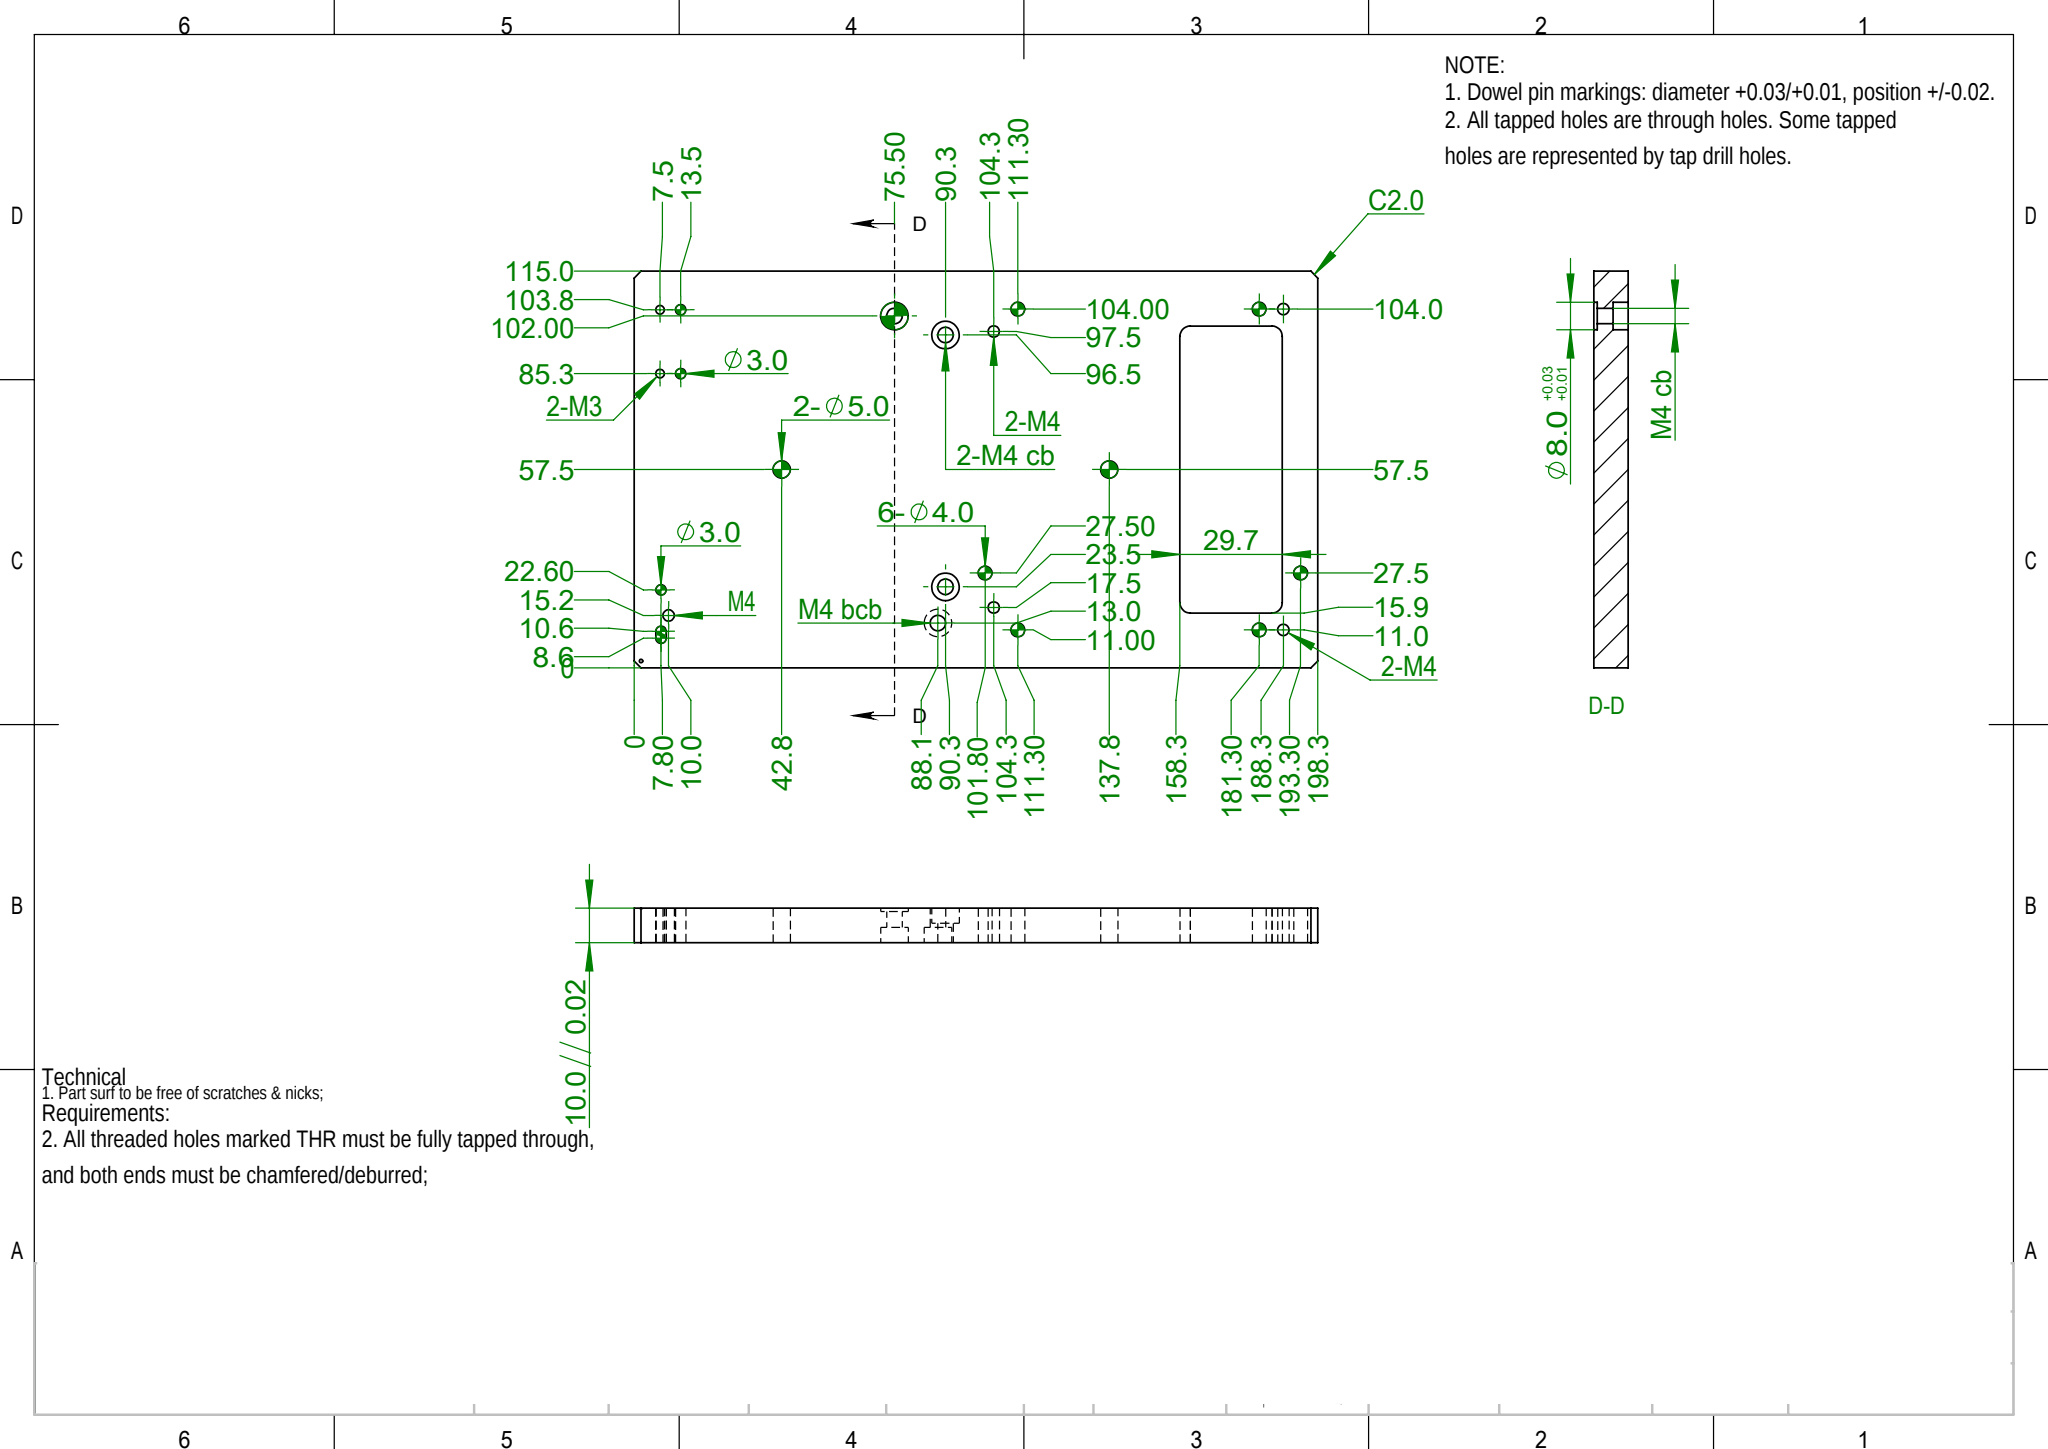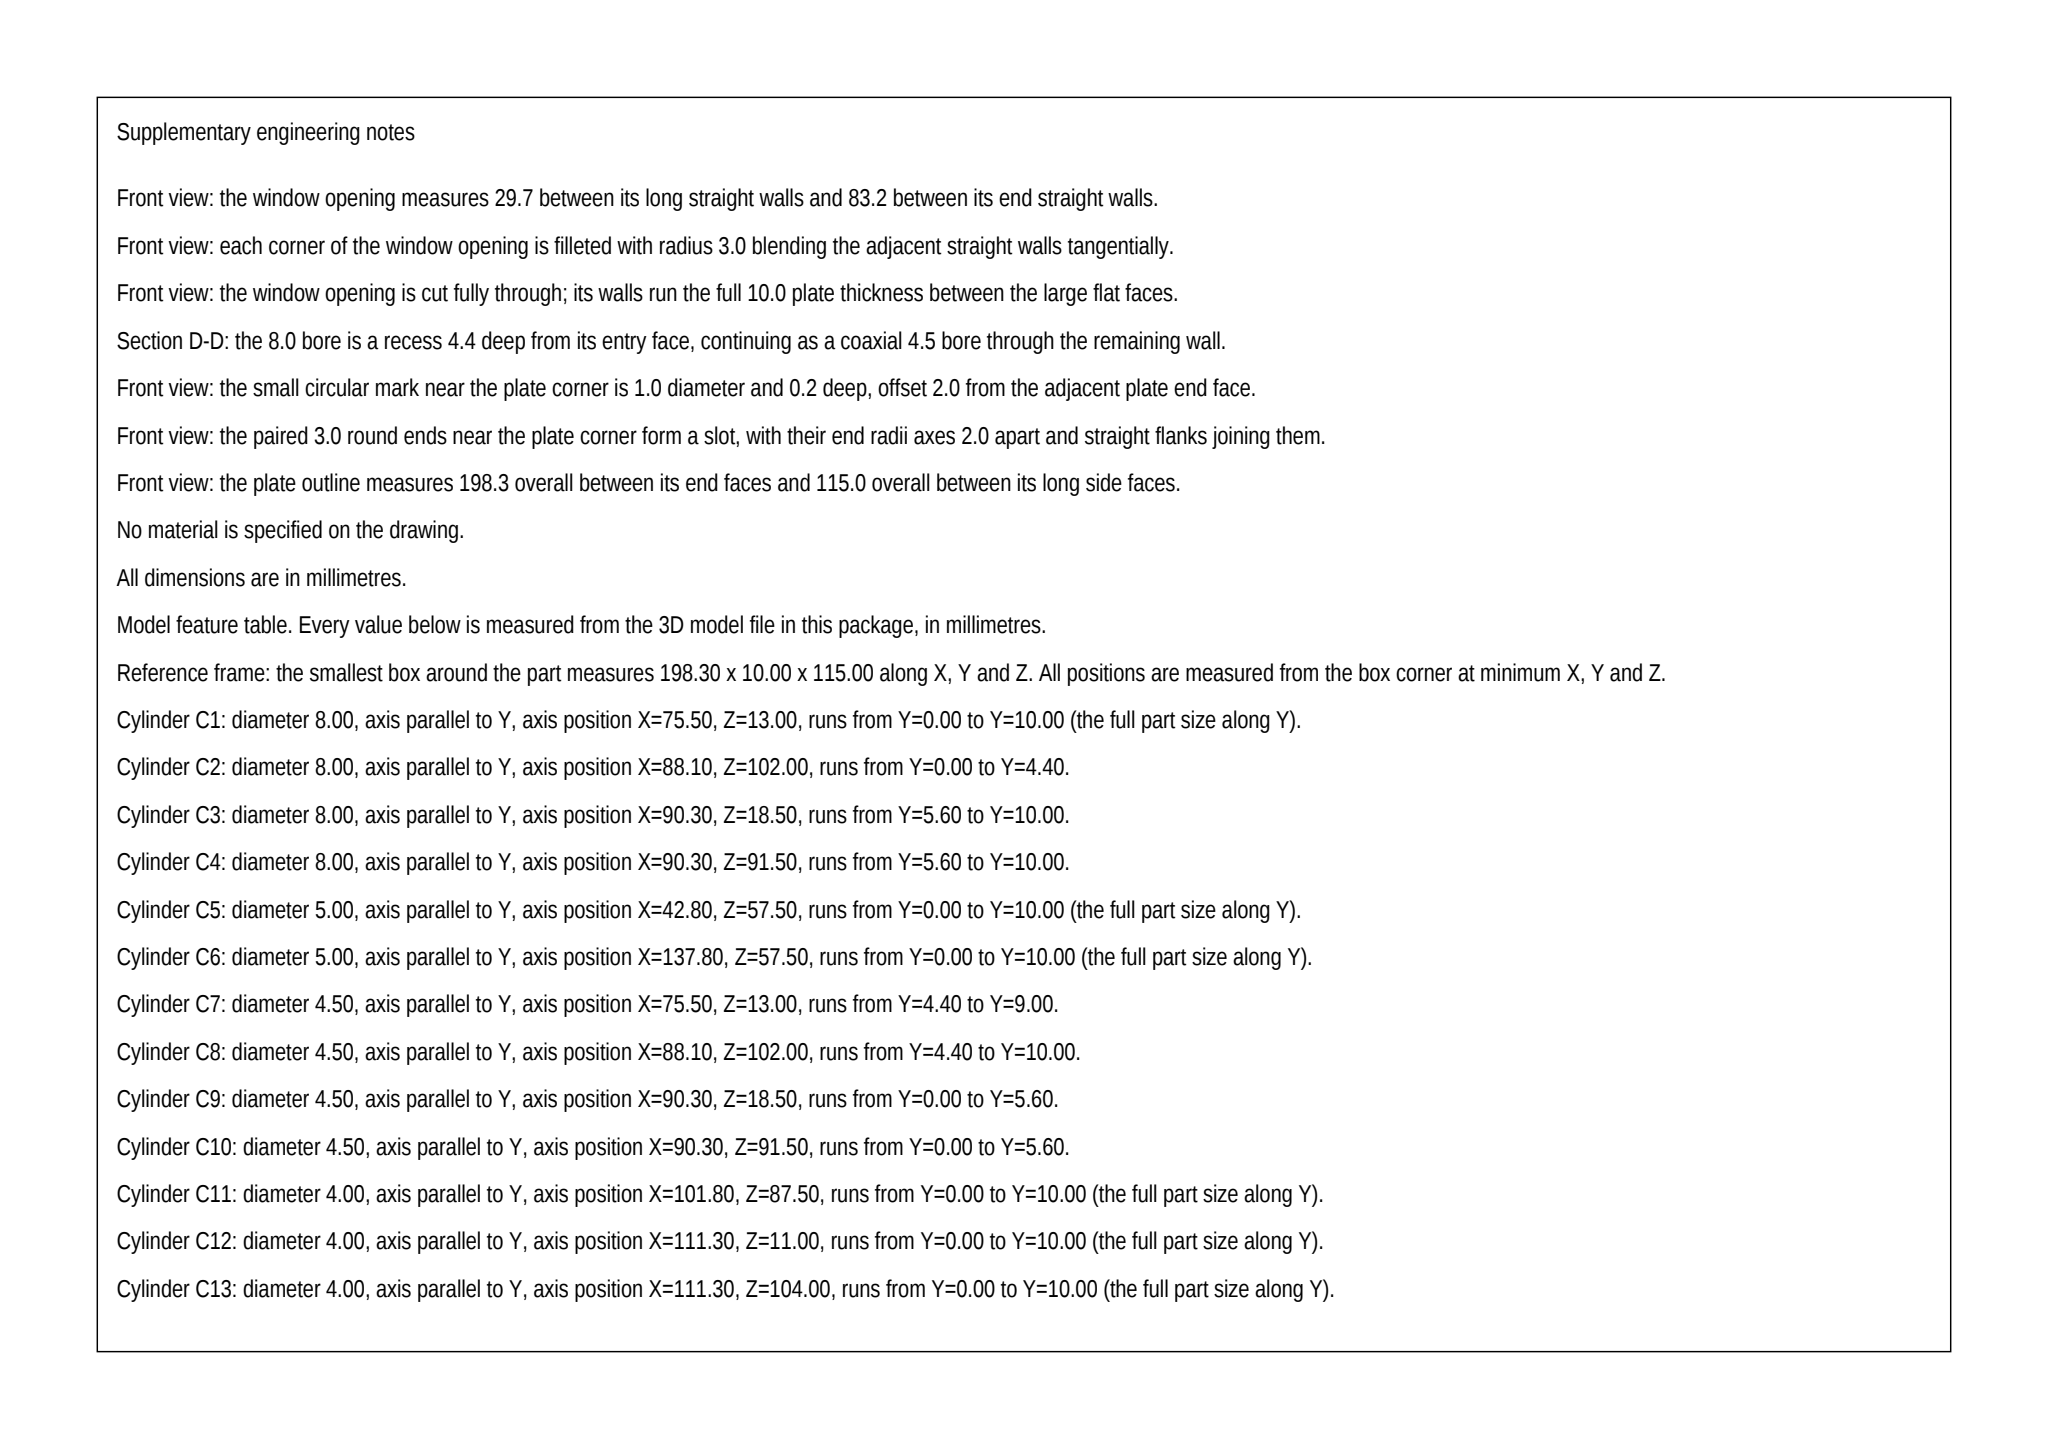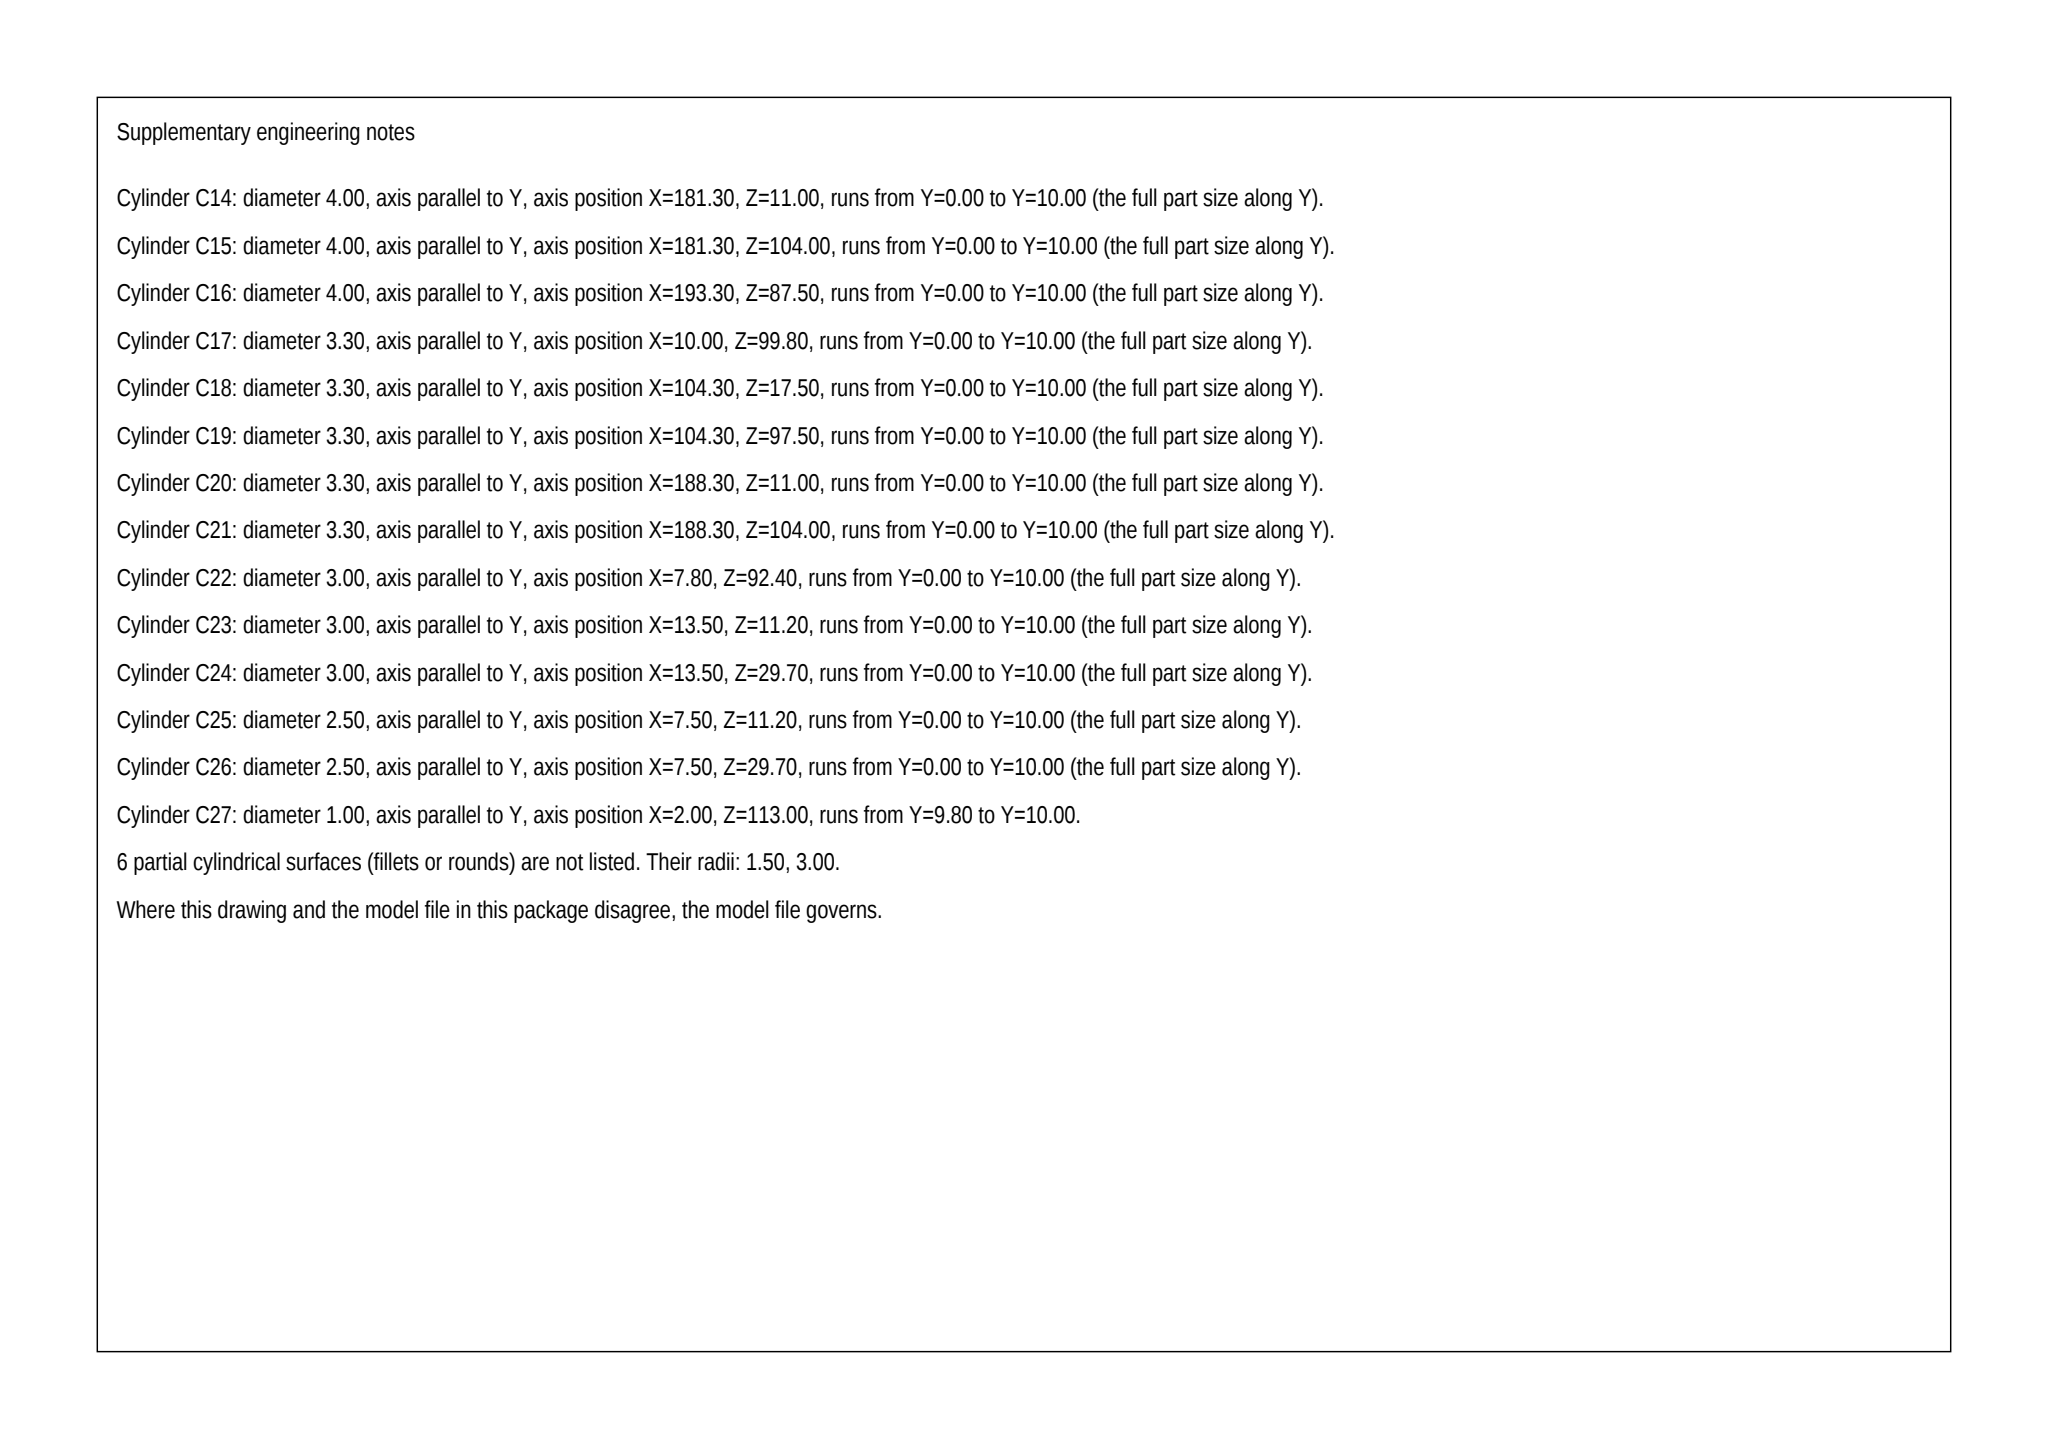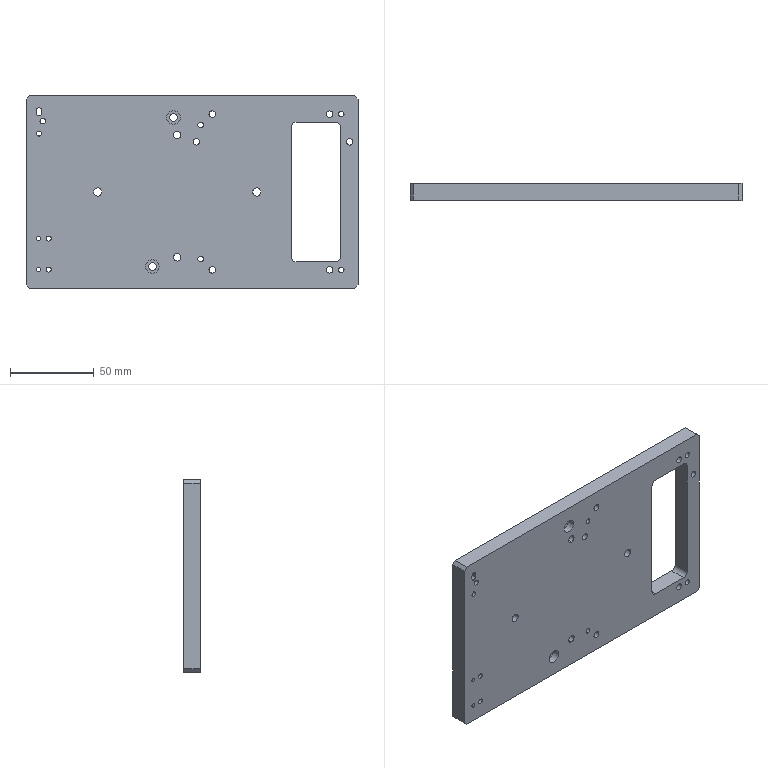Part | SolidWorks | mm | 1 solid | 84 faces | box 198.3 x 10 x 115 mm | volume 200041 mm3 | cylinder 62 | plane 22 | commonest cylinder face diameters 4 x12 8 x10 3.3 x10 4.5 x8 3 x8 5 x4 2.5 x4 6 x4
Drawing notes:
PLATE THK 10.0 - SEE SECT D-D | from the solid: bbox_xyz y = 10.0; planes y=0.0 and y=10.0
M4 CB & 2-M4 CB: Ø8.0 DP 4.4 | from the solid: cylinders [8.0,y,...,4.4] at (75.5,13.0),(88.1,102.0),(90.3,18.5),(90.3,91.5)
Ø1.0 DP 0.2 MARK: 2.0 FROM LH EDGE, 2.0 FROM TOP EDGE | from the solid: cylinder [1.0,y,[2.0,null,113.0],0.2]; bbox z=115.0, x=0 at LH edge
M4 cb/M4 bcb/2-M4 cb: Ø4.5 THRU, C'BORE Ø8.0 DP 4.4 | from the solid: Ø4.5 thru holes at x=88.1,90.3 (len 5.6) & x=75.5 (len 4.6) each with Ø8.0 x 4.4 deep c'bore; plate 10 thk
M4 bcb: ADD OPP SIDE C'BORE Ø8.0 DP 1.0 (SEE D-D) | from the solid: second Ø8.0 x 1.0 cylinder coaxial at [75.5,13.0] opposite the Ø8.0 x 4.4
29.7 X 83.2 CUTOUT, 4X R3.0: THRU (10 THK) | from the solid: x planes 158.3 & 188.0 (29.7), z planes 15.9 & 99.1 (83.2); bbox y = 10.0 thk, no floor face